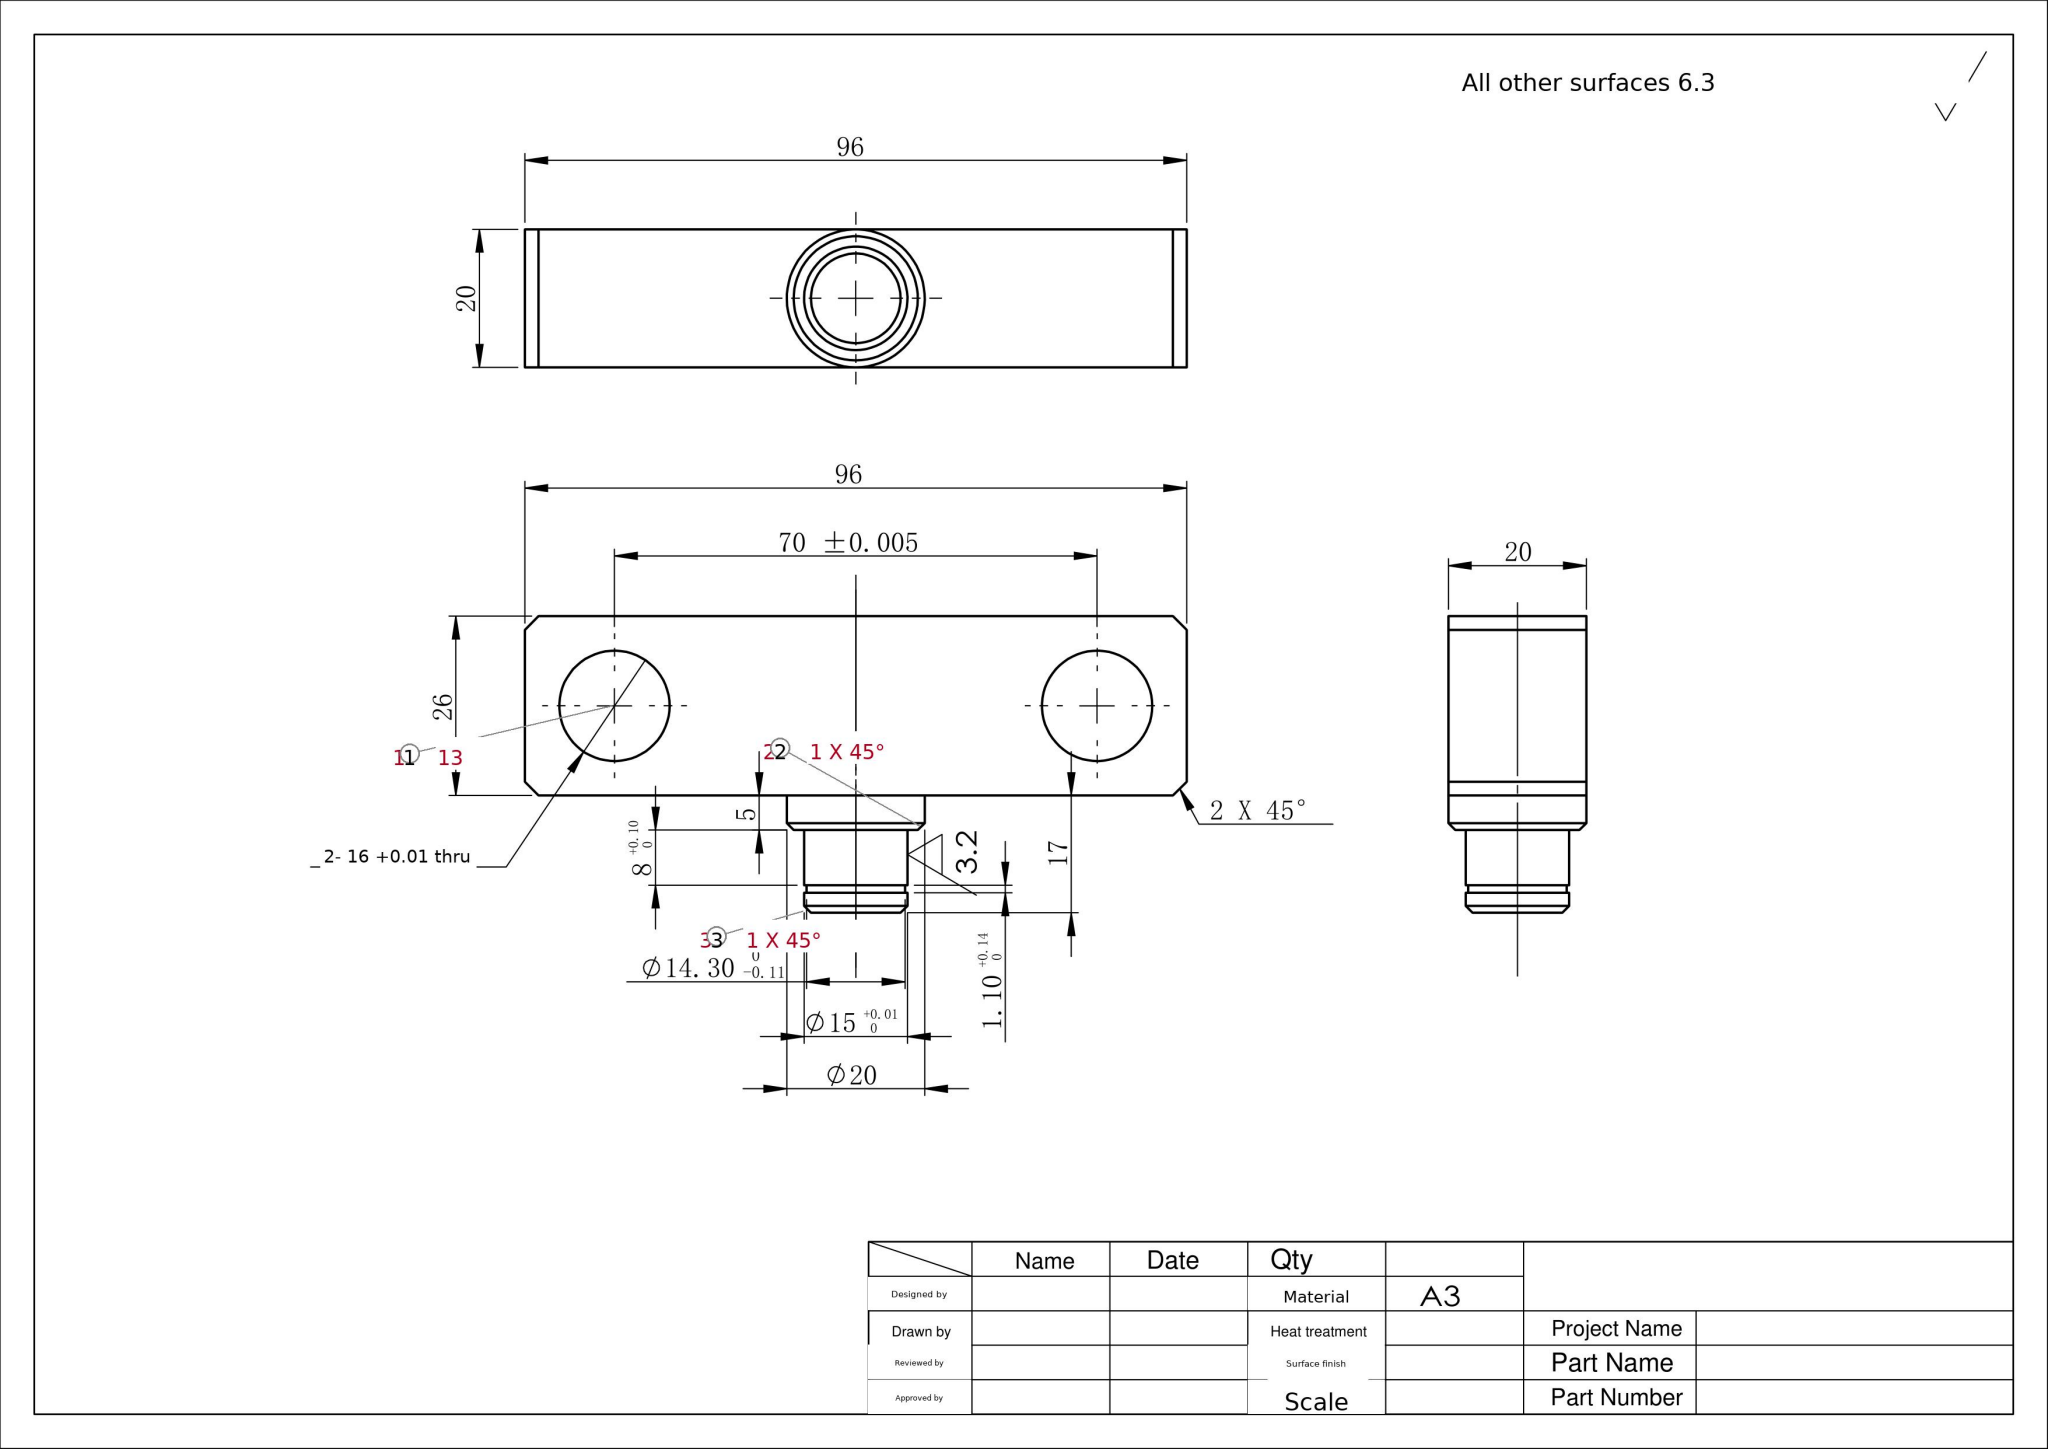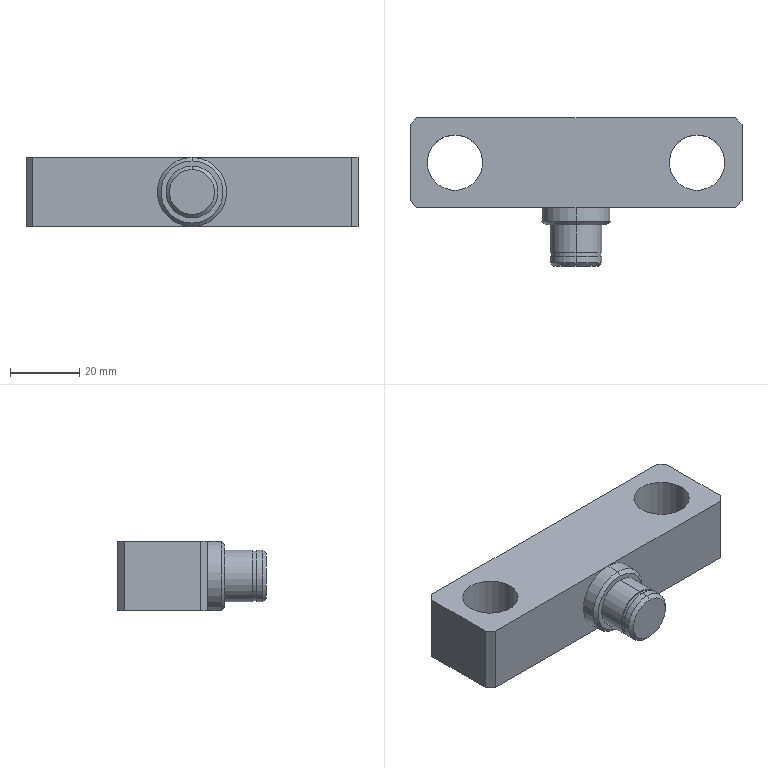Part | SolidWorks | mm | 1 solid | 31 faces | box 96 x 43 x 20 mm | volume 45338 mm3 | plane 15 | cylinder 12 | cone 4 | commonest cylinder face diameters 15 x4 16 x4 14.3 x2 20 x2
build123d program:
from build123d import *

# Parameters (mm, degrees)
SKETCH1_W      = 96
SKETCH1_H      = 26
SKETCH1_R      = 8
EXTRUDE1_DEPTH = 20
SKETCH2_R      = 10
EXTRUDE5_DEPTH = 5
SKETCH5_R      = 7.5
EXTRUDE6_DEPTH = 12
CHAMFER2_SIZE  = 1
SKETCH6_W      = 2.17
SKETCH6_H      = 1.1
CHAMFER3_SIZE  = 2


with BuildPart() as part:
    # Sketch1 → Extrude1 (new body)
    with BuildSketch(Plane.XY):
        with Locations((48, 13)):
            Rectangle(SKETCH1_W, SKETCH1_H)
        with Locations((13, 13)):
            Circle(SKETCH1_R, mode=Mode.SUBTRACT)
        with Locations((83, 13)):
            Circle(SKETCH1_R, mode=Mode.SUBTRACT)
    extrude(amount=EXTRUDE1_DEPTH)

    # Sketch2 → Extrude5 (add)
    with BuildSketch(Plane.XZ):
        with Locations(Location((48, 10, 0), (0, 0, 270))):
            Circle(SKETCH2_R)
    extrude(amount=EXTRUDE5_DEPTH)

    # Sketch5 → Extrude6 (add)
    with BuildSketch(Plane.XZ.offset(5)):
        with Locations(Location((48, 10, 0), (0, 0, 270))):
            Circle(SKETCH5_R)
    extrude(amount=EXTRUDE6_DEPTH)

    # Chamfer2
    chamfer2_edges = [part.edges().sort_by_distance(p)[0] for p in [
        (48, -5, 20),
        (48, -17, 17.5),
    ]]
    chamfer(chamfer2_edges, length=CHAMFER2_SIZE)

    # Sketch6 → Cut-Revolve1 (revolve, cut)
    with BuildSketch(Plane.XY.offset(10), mode=Mode.PRIVATE) as cut_revolve1_sk:
        with Locations((39.765, -13.55)):
            Rectangle(SKETCH6_W, SKETCH6_H)
    revolve(cut_revolve1_sk.sketch.rotate(Axis((48, -16, 10), (0, -1, 0)), 270), axis=Axis((48, -16, 10), (0, -1, 0)), mode=Mode.SUBTRACT)

    # Chamfer3
    chamfer3_edges = [part.edges().sort_by_distance(p)[0] for p in [
        (0, 26, 10),
        (96, 26, 10),
        (96, 0, 10),
        (0, 0, 10),
    ]]
    chamfer(chamfer3_edges, length=CHAMFER3_SIZE)


solid = part.part
STEP:
#1=CARTESIAN_POINT('',(48.,-16.,17.5));
#2=VERTEX_POINT('',#1);
#3=CARTESIAN_POINT('',(48.,-16.,2.5));
#4=VERTEX_POINT('',#3);
#5=CARTESIAN_POINT('',(48.,-16.,10.));
#6=DIRECTION('',(0.,1.,0.));
#7=DIRECTION('',(0.,0.,-1.));
#8=AXIS2_PLACEMENT_3D('',#5,#6,#7);
#9=CIRCLE('',#8,7.5);
#10=EDGE_CURVE('',#2,#4,#9,.T.);
#11=ORIENTED_EDGE('',*,*,#10,.T.);
#12=CARTESIAN_POINT('',(48.,-14.1,2.5));
#13=VERTEX_POINT('',#12);
#14=CARTESIAN_POINT('',(48.,-17.,2.5));
#15=DIRECTION('',(0.,1.,0.));
#16=VECTOR('',#15,1000.);
#17=LINE('',#14,#16);
#18=EDGE_CURVE('',#4,#13,#17,.T.);
#19=ORIENTED_EDGE('',*,*,#18,.T.);
#20=CARTESIAN_POINT('',(48.,-14.1,17.5));
#21=VERTEX_POINT('',#20);
#22=CARTESIAN_POINT('',(48.,-14.1,10.));
#23=DIRECTION('',(0.,-1.,0.));
#24=DIRECTION('',(0.,0.,-1.));
#25=AXIS2_PLACEMENT_3D('',#22,#23,#24);
#26=CIRCLE('',#25,7.5);
#27=EDGE_CURVE('',#13,#21,#26,.T.);
#28=ORIENTED_EDGE('',*,*,#27,.T.);
#29=CARTESIAN_POINT('',(48.,-17.,17.5));
#30=DIRECTION('',(0.,1.,0.));
#31=VECTOR('',#30,1000.);
#32=LINE('',#29,#31);
#33=EDGE_CURVE('',#2,#21,#32,.T.);
#34=ORIENTED_EDGE('',*,*,#33,.F.);
#35=EDGE_LOOP('',(#11,#19,#28,#34));
#36=FACE_OUTER_BOUND('',#35,.T.);
#37=CARTESIAN_POINT('',(48.,-17.,10.));
#38=DIRECTION('',(0.,1.,0.));
#39=DIRECTION('',(0.,0.,1.));
#40=AXIS2_PLACEMENT_3D('',#37,#38,#39);
#41=CYLINDRICAL_SURFACE('',#40,7.5);
#42=ADVANCED_FACE('',(#36),#41,.T.);
#43=CARTESIAN_POINT('',(48.,-17.,3.5));
#44=VERTEX_POINT('',#43);
#45=CARTESIAN_POINT('',(48.,-17.,16.5));
#46=VERTEX_POINT('',#45);
#47=CARTESIAN_POINT('',(48.,-17.,10.));
#48=DIRECTION('',(0.,-1.,0.));
#49=DIRECTION('',(0.,0.,-1.));
#50=AXIS2_PLACEMENT_3D('',#47,#48,#49);
#51=CIRCLE('',#50,6.5);
#52=EDGE_CURVE('',#44,#46,#51,.T.);
#53=ORIENTED_EDGE('',*,*,#52,.F.);
#54=CARTESIAN_POINT('',(48.,-17.,3.5));
#55=DIRECTION('',(0.,0.7071,-0.7071));
#56=VECTOR('',#55,1000.);
#57=LINE('',#54,#56);
#58=EDGE_CURVE('',#44,#4,#57,.T.);
#59=ORIENTED_EDGE('',*,*,#58,.T.);
#60=ORIENTED_EDGE('',*,*,#10,.F.);
#61=CARTESIAN_POINT('',(48.,-17.,16.5));
#62=DIRECTION('',(0.,0.7071,0.7071));
#63=VECTOR('',#62,1000.);
#64=LINE('',#61,#63);
#65=EDGE_CURVE('',#46,#2,#64,.T.);
#66=ORIENTED_EDGE('',*,*,#65,.F.);
#67=EDGE_LOOP('',(#53,#59,#60,#66));
#68=FACE_OUTER_BOUND('',#67,.T.);
#69=CARTESIAN_POINT('',(48.,-17.,10.));
#70=DIRECTION('',(0.,1.,0.));
#71=DIRECTION('',(0.,0.,1.));
#72=AXIS2_PLACEMENT_3D('',#69,#70,#71);
#73=CONICAL_SURFACE('',#72,6.5,0.7854);
#74=ADVANCED_FACE('',(#68),#73,.T.);
#75=CARTESIAN_POINT('',(48.,-14.1,17.15));
#76=VERTEX_POINT('',#75);
#77=CARTESIAN_POINT('',(48.,-14.1,2.85));
#78=VERTEX_POINT('',#77);
#79=CARTESIAN_POINT('',(48.,-14.1,10.));
#80=DIRECTION('',(0.,1.,0.));
#81=DIRECTION('',(0.,0.,1.));
#82=AXIS2_PLACEMENT_3D('',#79,#80,#81);
#83=CIRCLE('',#82,7.15);
#84=EDGE_CURVE('',#76,#78,#83,.T.);
#85=ORIENTED_EDGE('',*,*,#84,.T.);
#86=CARTESIAN_POINT('',(48.,-13.,2.85));
#87=VERTEX_POINT('',#86);
#88=CARTESIAN_POINT('',(48.,-16.,2.85));
#89=DIRECTION('',(0.,1.,0.));
#90=VECTOR('',#89,1000.);
#91=LINE('',#88,#90);
#92=EDGE_CURVE('',#78,#87,#91,.T.);
#93=ORIENTED_EDGE('',*,*,#92,.T.);
#94=CARTESIAN_POINT('',(48.,-13.,17.15));
#95=VERTEX_POINT('',#94);
#96=CARTESIAN_POINT('',(48.,-13.,10.));
#97=DIRECTION('',(0.,1.,0.));
#98=DIRECTION('',(0.,0.,1.));
#99=AXIS2_PLACEMENT_3D('',#96,#97,#98);
#100=CIRCLE('',#99,7.15);
#101=EDGE_CURVE('',#95,#87,#100,.T.);
#102=ORIENTED_EDGE('',*,*,#101,.F.);
#103=CARTESIAN_POINT('',(48.,-16.,17.15));
#104=DIRECTION('',(0.,1.,0.));
#105=VECTOR('',#104,1000.);
#106=LINE('',#103,#105);
#107=EDGE_CURVE('',#76,#95,#106,.T.);
#108=ORIENTED_EDGE('',*,*,#107,.F.);
#109=EDGE_LOOP('',(#85,#93,#102,#108));
#110=FACE_OUTER_BOUND('',#109,.T.);
#111=CARTESIAN_POINT('',(48.,-16.,10.));
#112=DIRECTION('',(0.,1.,0.));
#113=DIRECTION('',(0.,0.,1.));
#114=AXIS2_PLACEMENT_3D('',#111,#112,#113);
#115=CYLINDRICAL_SURFACE('',#114,7.15);
#116=ADVANCED_FACE('',(#110),#115,.T.);
#117=CARTESIAN_POINT('',(48.,-5.,1.));
#118=VERTEX_POINT('',#117);
#119=CARTESIAN_POINT('',(48.,-5.,19.));
#120=VERTEX_POINT('',#119);
#121=CARTESIAN_POINT('',(48.,-5.,10.));
#122=DIRECTION('',(0.,-1.,0.));
#123=DIRECTION('',(0.,0.,-1.));
#124=AXIS2_PLACEMENT_3D('',#121,#122,#123);
#125=CIRCLE('',#124,9.);
#126=EDGE_CURVE('',#118,#120,#125,.T.);
#127=ORIENTED_EDGE('',*,*,#126,.F.);
#128=CARTESIAN_POINT('',(48.,-4.,-0.));
#129=VERTEX_POINT('',#128);
#130=CARTESIAN_POINT('',(48.,-5.,1.));
#131=DIRECTION('',(0.,0.7071,-0.7071));
#132=VECTOR('',#131,1000.);
#133=LINE('',#130,#132);
#134=EDGE_CURVE('',#118,#129,#133,.T.);
#135=ORIENTED_EDGE('',*,*,#134,.T.);
#136=CARTESIAN_POINT('',(48.,-4.,20.));
#137=VERTEX_POINT('',#136);
#138=CARTESIAN_POINT('',(48.,-4.,10.));
#139=DIRECTION('',(0.,1.,0.));
#140=DIRECTION('',(0.,0.,-1.));
#141=AXIS2_PLACEMENT_3D('',#138,#139,#140);
#142=CIRCLE('',#141,10.);
#143=EDGE_CURVE('',#137,#129,#142,.T.);
#144=ORIENTED_EDGE('',*,*,#143,.F.);
#145=CARTESIAN_POINT('',(48.,-5.,19.));
#146=DIRECTION('',(0.,0.7071,0.7071));
#147=VECTOR('',#146,1000.);
#148=LINE('',#145,#147);
#149=EDGE_CURVE('',#120,#137,#148,.T.);
#150=ORIENTED_EDGE('',*,*,#149,.F.);
#151=EDGE_LOOP('',(#127,#135,#144,#150));
#152=FACE_OUTER_BOUND('',#151,.T.);
#153=CARTESIAN_POINT('',(48.,-5.,10.));
#154=DIRECTION('',(0.,1.,0.));
#155=DIRECTION('',(0.,0.,1.));
#156=AXIS2_PLACEMENT_3D('',#153,#154,#155);
#157=CONICAL_SURFACE('',#156,9.,0.7854);
#158=ADVANCED_FACE('',(#152),#157,.T.);
#159=ORIENTED_EDGE('',*,*,#143,.T.);
#160=CARTESIAN_POINT('',(48.,0.,-0.));
#161=VERTEX_POINT('',#160);
#162=CARTESIAN_POINT('',(48.,-5.,-0.));
#163=DIRECTION('',(0.,1.,0.));
#164=VECTOR('',#163,1000.);
#165=LINE('',#162,#164);
#166=EDGE_CURVE('',#129,#161,#165,.T.);
#167=ORIENTED_EDGE('',*,*,#166,.T.);
#168=CARTESIAN_POINT('',(48.,0.,20.));
#169=VERTEX_POINT('',#168);
#170=CARTESIAN_POINT('',(48.,0.,10.));
#171=DIRECTION('',(0.,-1.,0.));
#172=DIRECTION('',(0.,0.,-1.));
#173=AXIS2_PLACEMENT_3D('',#170,#171,#172);
#174=CIRCLE('',#173,10.);
#175=EDGE_CURVE('',#161,#169,#174,.T.);
#176=ORIENTED_EDGE('',*,*,#175,.T.);
#177=CARTESIAN_POINT('',(48.,-5.,20.));
#178=DIRECTION('',(0.,1.,0.));
#179=VECTOR('',#178,1000.);
#180=LINE('',#177,#179);
#181=EDGE_CURVE('',#137,#169,#180,.T.);
#182=ORIENTED_EDGE('',*,*,#181,.F.);
#183=EDGE_LOOP('',(#159,#167,#176,#182));
#184=FACE_OUTER_BOUND('',#183,.T.);
#185=CARTESIAN_POINT('',(48.,-5.,10.));
#186=DIRECTION('',(0.,1.,0.));
#187=DIRECTION('',(0.,0.,1.));
#188=AXIS2_PLACEMENT_3D('',#185,#186,#187);
#189=CYLINDRICAL_SURFACE('',#188,10.);
#190=ADVANCED_FACE('',(#184),#189,.T.);
#191=CARTESIAN_POINT('',(75.,13.,20.));
#192=VERTEX_POINT('',#191);
#193=CARTESIAN_POINT('',(91.,13.,20.));
#194=VERTEX_POINT('',#193);
#195=CARTESIAN_POINT('',(83.,13.,20.));
#196=DIRECTION('',(0.,0.,1.));
#197=DIRECTION('',(1.,0.,0.));
#198=AXIS2_PLACEMENT_3D('',#195,#196,#197);
#199=CIRCLE('',#198,8.);
#200=EDGE_CURVE('',#192,#194,#199,.T.);
#201=ORIENTED_EDGE('',*,*,#200,.T.);
#202=CARTESIAN_POINT('',(91.,13.,0.));
#203=VERTEX_POINT('',#202);
#204=CARTESIAN_POINT('',(91.,13.,20.));
#205=DIRECTION('',(0.,0.,-1.));
#206=VECTOR('',#205,1000.);
#207=LINE('',#204,#206);
#208=EDGE_CURVE('',#194,#203,#207,.T.);
#209=ORIENTED_EDGE('',*,*,#208,.T.);
#210=CARTESIAN_POINT('',(75.,13.,0.));
#211=VERTEX_POINT('',#210);
#212=CARTESIAN_POINT('',(83.,13.,0.));
#213=DIRECTION('',(0.,0.,1.));
#214=DIRECTION('',(1.,0.,0.));
#215=AXIS2_PLACEMENT_3D('',#212,#213,#214);
#216=CIRCLE('',#215,8.);
#217=EDGE_CURVE('',#211,#203,#216,.T.);
#218=ORIENTED_EDGE('',*,*,#217,.F.);
#219=CARTESIAN_POINT('',(75.,13.,20.));
#220=DIRECTION('',(0.,0.,-1.));
#221=VECTOR('',#220,1000.);
#222=LINE('',#219,#221);
#223=EDGE_CURVE('',#192,#211,#222,.T.);
#224=ORIENTED_EDGE('',*,*,#223,.F.);
#225=EDGE_LOOP('',(#201,#209,#218,#224));
#226=FACE_OUTER_BOUND('',#225,.T.);
#227=CARTESIAN_POINT('',(83.,13.,20.));
#228=DIRECTION('',(0.,0.,-1.));
#229=DIRECTION('',(-1.,0.,0.));
#230=AXIS2_PLACEMENT_3D('',#227,#228,#229);
#231=CYLINDRICAL_SURFACE('',#230,8.);
#232=ADVANCED_FACE('',(#226),#231,.F.);
#233=CARTESIAN_POINT('',(5.,13.,20.));
#234=VERTEX_POINT('',#233);
#235=CARTESIAN_POINT('',(21.,13.,20.));
#236=VERTEX_POINT('',#235);
#237=CARTESIAN_POINT('',(13.,13.,20.));
#238=DIRECTION('',(0.,0.,1.));
#239=DIRECTION('',(1.,0.,0.));
#240=AXIS2_PLACEMENT_3D('',#237,#238,#239);
#241=CIRCLE('',#240,8.);
#242=EDGE_CURVE('',#234,#236,#241,.T.);
#243=ORIENTED_EDGE('',*,*,#242,.T.);
#244=CARTESIAN_POINT('',(21.,13.,0.));
#245=VERTEX_POINT('',#244);
#246=CARTESIAN_POINT('',(21.,13.,20.));
#247=DIRECTION('',(0.,0.,-1.));
#248=VECTOR('',#247,1000.);
#249=LINE('',#246,#248);
#250=EDGE_CURVE('',#236,#245,#249,.T.);
#251=ORIENTED_EDGE('',*,*,#250,.T.);
#252=CARTESIAN_POINT('',(5.,13.,0.));
#253=VERTEX_POINT('',#252);
#254=CARTESIAN_POINT('',(13.,13.,0.));
#255=DIRECTION('',(0.,0.,1.));
#256=DIRECTION('',(1.,0.,0.));
#257=AXIS2_PLACEMENT_3D('',#254,#255,#256);
#258=CIRCLE('',#257,8.);
#259=EDGE_CURVE('',#253,#245,#258,.T.);
#260=ORIENTED_EDGE('',*,*,#259,.F.);
#261=CARTESIAN_POINT('',(5.,13.,20.));
#262=DIRECTION('',(0.,0.,-1.));
#263=VECTOR('',#262,1000.);
#264=LINE('',#261,#263);
#265=EDGE_CURVE('',#234,#253,#264,.T.);
#266=ORIENTED_EDGE('',*,*,#265,.F.);
#267=EDGE_LOOP('',(#243,#251,#260,#266));
#268=FACE_OUTER_BOUND('',#267,.T.);
#269=CARTESIAN_POINT('',(13.,13.,20.));
#270=DIRECTION('',(0.,0.,-1.));
#271=DIRECTION('',(-1.,0.,0.));
#272=AXIS2_PLACEMENT_3D('',#269,#270,#271);
#273=CYLINDRICAL_SURFACE('',#272,8.);
#274=ADVANCED_FACE('',(#268),#273,.F.);
#275=CARTESIAN_POINT('',(48.,-13.,17.5));
#276=VERTEX_POINT('',#275);
#277=CARTESIAN_POINT('',(48.,-13.,2.5));
#278=VERTEX_POINT('',#277);
#279=CARTESIAN_POINT('',(48.,-13.,10.));
#280=DIRECTION('',(0.,1.,0.));
#281=DIRECTION('',(0.,0.,1.));
#282=AXIS2_PLACEMENT_3D('',#279,#280,#281);
#283=CIRCLE('',#282,7.5);
#284=EDGE_CURVE('',#276,#278,#283,.T.);
#285=ORIENTED_EDGE('',*,*,#284,.T.);
#286=CARTESIAN_POINT('',(48.,-5.,2.5));
#287=VERTEX_POINT('',#286);
#288=CARTESIAN_POINT('',(48.,-17.,2.5));
#289=DIRECTION('',(0.,1.,0.));
#290=VECTOR('',#289,1000.);
#291=LINE('',#288,#290);
#292=EDGE_CURVE('',#278,#287,#291,.T.);
#293=ORIENTED_EDGE('',*,*,#292,.T.);
#294=CARTESIAN_POINT('',(48.,-5.,17.5));
#295=VERTEX_POINT('',#294);
#296=CARTESIAN_POINT('',(48.,-5.,10.));
#297=DIRECTION('',(0.,-1.,0.));
#298=DIRECTION('',(0.,0.,-1.));
#299=AXIS2_PLACEMENT_3D('',#296,#297,#298);
#300=CIRCLE('',#299,7.5);
#301=EDGE_CURVE('',#287,#295,#300,.T.);
#302=ORIENTED_EDGE('',*,*,#301,.T.);
#303=CARTESIAN_POINT('',(48.,-17.,17.5));
#304=DIRECTION('',(0.,1.,0.));
#305=VECTOR('',#304,1000.);
#306=LINE('',#303,#305);
#307=EDGE_CURVE('',#276,#295,#306,.T.);
#308=ORIENTED_EDGE('',*,*,#307,.F.);
#309=EDGE_LOOP('',(#285,#293,#302,#308));
#310=FACE_OUTER_BOUND('',#309,.T.);
#311=CARTESIAN_POINT('',(48.,-17.,10.));
#312=DIRECTION('',(0.,1.,0.));
#313=DIRECTION('',(0.,0.,1.));
#314=AXIS2_PLACEMENT_3D('',#311,#312,#313);
#315=CYLINDRICAL_SURFACE('',#314,7.5);
#316=ADVANCED_FACE('',(#310),#315,.T.);
#317=ORIENTED_EDGE('',*,*,#292,.F.);
#318=CARTESIAN_POINT('',(48.,-13.,10.));
#319=DIRECTION('',(0.,1.,0.));
#320=DIRECTION('',(0.,0.,1.));
#321=AXIS2_PLACEMENT_3D('',#318,#319,#320);
#322=CIRCLE('',#321,7.5);
#323=EDGE_CURVE('',#278,#276,#322,.T.);
#324=ORIENTED_EDGE('',*,*,#323,.T.);
#325=ORIENTED_EDGE('',*,*,#307,.T.);
#326=CARTESIAN_POINT('',(48.,-5.,10.));
#327=DIRECTION('',(0.,-1.,0.));
#328=DIRECTION('',(0.,0.,-1.));
#329=AXIS2_PLACEMENT_3D('',#326,#327,#328);
#330=CIRCLE('',#329,7.5);
#331=EDGE_CURVE('',#295,#287,#330,.T.);
#332=ORIENTED_EDGE('',*,*,#331,.T.);
#333=EDGE_LOOP('',(#317,#324,#325,#332));
#334=FACE_OUTER_BOUND('',#333,.T.);
#335=CARTESIAN_POINT('',(48.,-17.,10.));
#336=DIRECTION('',(0.,1.,0.));
#337=DIRECTION('',(0.,0.,1.));
#338=AXIS2_PLACEMENT_3D('',#335,#336,#337);
#339=CYLINDRICAL_SURFACE('',#338,7.5);
#340=ADVANCED_FACE('',(#334),#339,.T.);
#341=CARTESIAN_POINT('',(48.,-5.,10.));
#342=DIRECTION('',(0.,-1.,0.));
#343=DIRECTION('',(0.,0.,-1.));
#344=AXIS2_PLACEMENT_3D('',#341,#342,#343);
#345=CIRCLE('',#344,9.);
#346=EDGE_CURVE('',#120,#118,#345,.T.);
#347=ORIENTED_EDGE('',*,*,#346,.T.);
#348=ORIENTED_EDGE('',*,*,#126,.T.);
#349=EDGE_LOOP('',(#347,#348));
#350=FACE_OUTER_BOUND('',#349,.T.);
#351=ORIENTED_EDGE('',*,*,#331,.F.);
#352=ORIENTED_EDGE('',*,*,#301,.F.);
#353=EDGE_LOOP('',(#351,#352));
#354=FACE_BOUND('',#353,.T.);
#355=CARTESIAN_POINT('',(48.,-5.,10.));
#356=DIRECTION('',(0.,-1.,0.));
#357=DIRECTION('',(0.,0.,-1.));
#358=AXIS2_PLACEMENT_3D('',#355,#356,#357);
#359=PLANE('',#358);
#360=ADVANCED_FACE('',(#350,#354),#359,.T.);
#361=CARTESIAN_POINT('',(94.,0.,0.));
#362=VERTEX_POINT('',#361);
#363=CARTESIAN_POINT('',(0.,0.,0.));
#364=DIRECTION('',(1.,0.,0.));
#365=VECTOR('',#364,1000.);
#366=LINE('',#363,#365);
#367=EDGE_CURVE('',#161,#362,#366,.T.);
#368=ORIENTED_EDGE('',*,*,#367,.T.);
#369=CARTESIAN_POINT('',(94.,-0.,20.));
#370=VERTEX_POINT('',#369);
#371=CARTESIAN_POINT('',(94.,0.,20.));
#372=DIRECTION('',(0.,0.,1.));
#373=VECTOR('',#372,1000.);
#374=LINE('',#371,#373);
#375=EDGE_CURVE('',#362,#370,#374,.T.);
#376=ORIENTED_EDGE('',*,*,#375,.T.);
#377=CARTESIAN_POINT('',(0.,0.,20.));
#378=DIRECTION('',(1.,0.,0.));
#379=VECTOR('',#378,1000.);
#380=LINE('',#377,#379);
#381=EDGE_CURVE('',#169,#370,#380,.T.);
#382=ORIENTED_EDGE('',*,*,#381,.F.);
#383=ORIENTED_EDGE('',*,*,#175,.F.);
#384=EDGE_LOOP('',(#368,#376,#382,#383));
#385=FACE_OUTER_BOUND('',#384,.T.);
#386=CARTESIAN_POINT('',(0.,0.,20.));
#387=DIRECTION('',(0.,1.,0.));
#388=DIRECTION('',(0.,0.,1.));
#389=AXIS2_PLACEMENT_3D('',#386,#387,#388);
#390=PLANE('',#389);
#391=ADVANCED_FACE('',(#385),#390,.F.);
#392=CARTESIAN_POINT('',(2.,0.,20.));
#393=VERTEX_POINT('',#392);
#394=CARTESIAN_POINT('',(0.,0.,20.));
#395=DIRECTION('',(1.,0.,0.));
#396=VECTOR('',#395,1000.);
#397=LINE('',#394,#396);
#398=EDGE_CURVE('',#393,#169,#397,.T.);
#399=ORIENTED_EDGE('',*,*,#398,.F.);
#400=CARTESIAN_POINT('',(2.,0.,0.));
#401=VERTEX_POINT('',#400);
#402=CARTESIAN_POINT('',(2.,0.,20.));
#403=DIRECTION('',(0.,0.,-1.));
#404=VECTOR('',#403,1000.);
#405=LINE('',#402,#404);
#406=EDGE_CURVE('',#393,#401,#405,.T.);
#407=ORIENTED_EDGE('',*,*,#406,.T.);
#408=CARTESIAN_POINT('',(0.,0.,0.));
#409=DIRECTION('',(1.,0.,0.));
#410=VECTOR('',#409,1000.);
#411=LINE('',#408,#410);
#412=EDGE_CURVE('',#401,#161,#411,.T.);
#413=ORIENTED_EDGE('',*,*,#412,.T.);
#414=CARTESIAN_POINT('',(48.,0.,10.));
#415=DIRECTION('',(0.,-1.,0.));
#416=DIRECTION('',(0.,0.,-1.));
#417=AXIS2_PLACEMENT_3D('',#414,#415,#416);
#418=CIRCLE('',#417,10.);
#419=EDGE_CURVE('',#169,#161,#418,.T.);
#420=ORIENTED_EDGE('',*,*,#419,.F.);
#421=EDGE_LOOP('',(#399,#407,#413,#420));
#422=FACE_OUTER_BOUND('',#421,.T.);
#423=CARTESIAN_POINT('',(0.,0.,20.));
#424=DIRECTION('',(0.,1.,0.));
#425=DIRECTION('',(0.,0.,1.));
#426=AXIS2_PLACEMENT_3D('',#423,#424,#425);
#427=PLANE('',#426);
#428=ADVANCED_FACE('',(#422),#427,.F.);
#429=ORIENTED_EDGE('',*,*,#242,.F.);
#430=CARTESIAN_POINT('',(13.,13.,20.));
#431=DIRECTION('',(0.,0.,1.));
#432=DIRECTION('',(1.,0.,0.));
#433=AXIS2_PLACEMENT_3D('',#430,#431,#432);
#434=CIRCLE('',#433,8.);
#435=EDGE_CURVE('',#236,#234,#434,.T.);
#436=ORIENTED_EDGE('',*,*,#435,.F.);
#437=EDGE_LOOP('',(#429,#436));
#438=FACE_BOUND('',#437,.T.);
#439=CARTESIAN_POINT('',(96.,2.,20.));
#440=VERTEX_POINT('',#439);
#441=CARTESIAN_POINT('',(96.,24.,20.));
#442=VERTEX_POINT('',#441);
#443=CARTESIAN_POINT('',(96.,0.,20.));
#444=DIRECTION('',(0.,1.,0.));
#445=VECTOR('',#444,1000.);
#446=LINE('',#443,#445);
#447=EDGE_CURVE('',#440,#442,#446,.T.);
#448=ORIENTED_EDGE('',*,*,#447,.T.);
#449=CARTESIAN_POINT('',(94.,26.,20.));
#450=VERTEX_POINT('',#449);
#451=CARTESIAN_POINT('',(94.,26.,20.));
#452=DIRECTION('',(-0.7071,0.7071,0.));
#453=VECTOR('',#452,1000.);
#454=LINE('',#451,#453);
#455=EDGE_CURVE('',#442,#450,#454,.T.);
#456=ORIENTED_EDGE('',*,*,#455,.T.);
#457=CARTESIAN_POINT('',(2.,26.,20.));
#458=VERTEX_POINT('',#457);
#459=CARTESIAN_POINT('',(0.,26.,20.));
#460=DIRECTION('',(-1.,0.,0.));
#461=VECTOR('',#460,1000.);
#462=LINE('',#459,#461);
#463=EDGE_CURVE('',#450,#458,#462,.T.);
#464=ORIENTED_EDGE('',*,*,#463,.T.);
#465=CARTESIAN_POINT('',(-0.,24.,20.));
#466=VERTEX_POINT('',#465);
#467=CARTESIAN_POINT('',(0.,24.,20.));
#468=DIRECTION('',(-0.7071,-0.7071,0.));
#469=VECTOR('',#468,1000.);
#470=LINE('',#467,#469);
#471=EDGE_CURVE('',#458,#466,#470,.T.);
#472=ORIENTED_EDGE('',*,*,#471,.T.);
#473=CARTESIAN_POINT('',(-0.,2.,20.));
#474=VERTEX_POINT('',#473);
#475=CARTESIAN_POINT('',(0.,0.,20.));
#476=DIRECTION('',(0.,-1.,0.));
#477=VECTOR('',#476,1000.);
#478=LINE('',#475,#477);
#479=EDGE_CURVE('',#466,#474,#478,.T.);
#480=ORIENTED_EDGE('',*,*,#479,.T.);
#481=CARTESIAN_POINT('',(2.,0.,20.));
#482=DIRECTION('',(0.7071,-0.7071,0.));
#483=VECTOR('',#482,1000.);
#484=LINE('',#481,#483);
#485=EDGE_CURVE('',#474,#393,#484,.T.);
#486=ORIENTED_EDGE('',*,*,#485,.T.);
#487=ORIENTED_EDGE('',*,*,#398,.T.);
#488=ORIENTED_EDGE('',*,*,#381,.T.);
#489=CARTESIAN_POINT('',(96.,2.,20.));
#490=DIRECTION('',(0.7071,0.7071,0.));
#491=VECTOR('',#490,1000.);
#492=LINE('',#489,#491);
#493=EDGE_CURVE('',#370,#440,#492,.T.);
#494=ORIENTED_EDGE('',*,*,#493,.T.);
#495=EDGE_LOOP('',(#448,#456,#464,#472,#480,#486,#487,#488,#494));
#496=FACE_OUTER_BOUND('',#495,.T.);
#497=ORIENTED_EDGE('',*,*,#200,.F.);
#498=CARTESIAN_POINT('',(83.,13.,20.));
#499=DIRECTION('',(0.,0.,1.));
#500=DIRECTION('',(1.,0.,0.));
#501=AXIS2_PLACEMENT_3D('',#498,#499,#500);
#502=CIRCLE('',#501,8.);
#503=EDGE_CURVE('',#194,#192,#502,.T.);
#504=ORIENTED_EDGE('',*,*,#503,.F.);
#505=EDGE_LOOP('',(#497,#504));
#506=FACE_BOUND('',#505,.T.);
#507=CARTESIAN_POINT('',(0.,0.,20.));
#508=DIRECTION('',(0.,0.,-1.));
#509=DIRECTION('',(-1.,0.,0.));
#510=AXIS2_PLACEMENT_3D('',#507,#508,#509);
#511=PLANE('',#510);
#512=ADVANCED_FACE('',(#438,#496,#506),#511,.F.);
#513=ORIENTED_EDGE('',*,*,#259,.T.);
#514=CARTESIAN_POINT('',(13.,13.,0.));
#515=DIRECTION('',(0.,0.,1.));
#516=DIRECTION('',(1.,0.,0.));
#517=AXIS2_PLACEMENT_3D('',#514,#515,#516);
#518=CIRCLE('',#517,8.);
#519=EDGE_CURVE('',#245,#253,#518,.T.);
#520=ORIENTED_EDGE('',*,*,#519,.T.);
#521=EDGE_LOOP('',(#513,#520));
#522=FACE_BOUND('',#521,.T.);
#523=CARTESIAN_POINT('',(94.,26.,0.));
#524=VERTEX_POINT('',#523);
#525=CARTESIAN_POINT('',(2.,26.,0.));
#526=VERTEX_POINT('',#525);
#527=CARTESIAN_POINT('',(0.,26.,0.));
#528=DIRECTION('',(-1.,0.,0.));
#529=VECTOR('',#528,1000.);
#530=LINE('',#527,#529);
#531=EDGE_CURVE('',#524,#526,#530,.T.);
#532=ORIENTED_EDGE('',*,*,#531,.F.);
#533=CARTESIAN_POINT('',(96.,24.,0.));
#534=VERTEX_POINT('',#533);
#535=CARTESIAN_POINT('',(60.,60.,0.));
#536=DIRECTION('',(0.7071,-0.7071,0.));
#537=VECTOR('',#536,1000.);
#538=LINE('',#535,#537);
#539=EDGE_CURVE('',#524,#534,#538,.T.);
#540=ORIENTED_EDGE('',*,*,#539,.T.);
#541=CARTESIAN_POINT('',(96.,2.,0.));
#542=VERTEX_POINT('',#541);
#543=CARTESIAN_POINT('',(96.,0.,0.));
#544=DIRECTION('',(0.,1.,0.));
#545=VECTOR('',#544,1000.);
#546=LINE('',#543,#545);
#547=EDGE_CURVE('',#542,#534,#546,.T.);
#548=ORIENTED_EDGE('',*,*,#547,.F.);
#549=CARTESIAN_POINT('',(47.,-47.,0.));
#550=DIRECTION('',(-0.7071,-0.7071,0.));
#551=VECTOR('',#550,1000.);
#552=LINE('',#549,#551);
#553=EDGE_CURVE('',#542,#362,#552,.T.);
#554=ORIENTED_EDGE('',*,*,#553,.T.);
#555=ORIENTED_EDGE('',*,*,#367,.F.);
#556=ORIENTED_EDGE('',*,*,#412,.F.);
#557=CARTESIAN_POINT('',(0.,2.,0.));
#558=VERTEX_POINT('',#557);
#559=CARTESIAN_POINT('',(1.,1.,0.));
#560=DIRECTION('',(-0.7071,0.7071,0.));
#561=VECTOR('',#560,1000.);
#562=LINE('',#559,#561);
#563=EDGE_CURVE('',#401,#558,#562,.T.);
#564=ORIENTED_EDGE('',*,*,#563,.T.);
#565=CARTESIAN_POINT('',(0.,24.,0.));
#566=VERTEX_POINT('',#565);
#567=CARTESIAN_POINT('',(0.,0.,0.));
#568=DIRECTION('',(0.,-1.,0.));
#569=VECTOR('',#568,1000.);
#570=LINE('',#567,#569);
#571=EDGE_CURVE('',#566,#558,#570,.T.);
#572=ORIENTED_EDGE('',*,*,#571,.F.);
#573=CARTESIAN_POINT('',(-12.,12.,0.));
#574=DIRECTION('',(0.7071,0.7071,0.));
#575=VECTOR('',#574,1000.);
#576=LINE('',#573,#575);
#577=EDGE_CURVE('',#566,#526,#576,.T.);
#578=ORIENTED_EDGE('',*,*,#577,.T.);
#579=EDGE_LOOP('',(#532,#540,#548,#554,#555,#556,#564,#572,#578));
#580=FACE_OUTER_BOUND('',#579,.T.);
#581=ORIENTED_EDGE('',*,*,#217,.T.);
#582=CARTESIAN_POINT('',(83.,13.,0.));
#583=DIRECTION('',(0.,0.,1.));
#584=DIRECTION('',(1.,0.,0.));
#585=AXIS2_PLACEMENT_3D('',#582,#583,#584);
#586=CIRCLE('',#585,8.);
#587=EDGE_CURVE('',#203,#211,#586,.T.);
#588=ORIENTED_EDGE('',*,*,#587,.T.);
#589=EDGE_LOOP('',(#581,#588));
#590=FACE_BOUND('',#589,.T.);
#591=CARTESIAN_POINT('',(0.,0.,0.));
#592=DIRECTION('',(0.,0.,-1.));
#593=DIRECTION('',(-1.,0.,0.));
#594=AXIS2_PLACEMENT_3D('',#591,#592,#593);
#595=PLANE('',#594);
#596=ADVANCED_FACE('',(#522,#580,#590),#595,.T.);
#597=ORIENTED_EDGE('',*,*,#479,.F.);
#598=CARTESIAN_POINT('',(0.,24.,20.));
#599=DIRECTION('',(0.,0.,-1.));
#600=VECTOR('',#599,1000.);
#601=LINE('',#598,#600);
#602=EDGE_CURVE('',#466,#566,#601,.T.);
#603=ORIENTED_EDGE('',*,*,#602,.T.);
#604=ORIENTED_EDGE('',*,*,#571,.T.);
#605=CARTESIAN_POINT('',(0.,2.,20.));
#606=DIRECTION('',(0.,0.,1.));
#607=VECTOR('',#606,1000.);
#608=LINE('',#605,#607);
#609=EDGE_CURVE('',#558,#474,#608,.T.);
#610=ORIENTED_EDGE('',*,*,#609,.T.);
#611=EDGE_LOOP('',(#597,#603,#604,#610));
#612=FACE_OUTER_BOUND('',#611,.T.);
#613=CARTESIAN_POINT('',(0.,0.,20.));
#614=DIRECTION('',(1.,0.,0.));
#615=DIRECTION('',(0.,0.,-1.));
#616=AXIS2_PLACEMENT_3D('',#613,#614,#615);
#617=PLANE('',#616);
#618=ADVANCED_FACE('',(#612),#617,.F.);
#619=ORIENTED_EDGE('',*,*,#547,.T.);
#620=CARTESIAN_POINT('',(96.,24.,20.));
#621=DIRECTION('',(0.,0.,1.));
#622=VECTOR('',#621,1000.);
#623=LINE('',#620,#622);
#624=EDGE_CURVE('',#534,#442,#623,.T.);
#625=ORIENTED_EDGE('',*,*,#624,.T.);
#626=ORIENTED_EDGE('',*,*,#447,.F.);
#627=CARTESIAN_POINT('',(96.,2.,20.));
#628=DIRECTION('',(0.,0.,-1.));
#629=VECTOR('',#628,1000.);
#630=LINE('',#627,#629);
#631=EDGE_CURVE('',#440,#542,#630,.T.);
#632=ORIENTED_EDGE('',*,*,#631,.T.);
#633=EDGE_LOOP('',(#619,#625,#626,#632));
#634=FACE_OUTER_BOUND('',#633,.T.);
#635=CARTESIAN_POINT('',(96.,0.,20.));
#636=DIRECTION('',(-1.,0.,0.));
#637=DIRECTION('',(0.,0.,1.));
#638=AXIS2_PLACEMENT_3D('',#635,#636,#637);
#639=PLANE('',#638);
#640=ADVANCED_FACE('',(#634),#639,.F.);
#641=ORIENTED_EDGE('',*,*,#463,.F.);
#642=CARTESIAN_POINT('',(94.,26.,20.));
#643=DIRECTION('',(0.,0.,-1.));
#644=VECTOR('',#643,1000.);
#645=LINE('',#642,#644);
#646=EDGE_CURVE('',#450,#524,#645,.T.);
#647=ORIENTED_EDGE('',*,*,#646,.T.);
#648=ORIENTED_EDGE('',*,*,#531,.T.);
#649=CARTESIAN_POINT('',(2.,26.,20.));
#650=DIRECTION('',(0.,0.,1.));
#651=VECTOR('',#650,1000.);
#652=LINE('',#649,#651);
#653=EDGE_CURVE('',#526,#458,#652,.T.);
#654=ORIENTED_EDGE('',*,*,#653,.T.);
#655=EDGE_LOOP('',(#641,#647,#648,#654));
#656=FACE_OUTER_BOUND('',#655,.T.);
#657=CARTESIAN_POINT('',(0.,26.,20.));
#658=DIRECTION('',(-0.,-1.,0.));
#659=DIRECTION('',(1.,-0.,0.));
#660=AXIS2_PLACEMENT_3D('',#657,#658,#659);
#661=PLANE('',#660);
#662=ADVANCED_FACE('',(#656),#661,.F.);
#663=ORIENTED_EDGE('',*,*,#250,.F.);
#664=ORIENTED_EDGE('',*,*,#435,.T.);
#665=ORIENTED_EDGE('',*,*,#265,.T.);
#666=ORIENTED_EDGE('',*,*,#519,.F.);
#667=EDGE_LOOP('',(#663,#664,#665,#666));
#668=FACE_OUTER_BOUND('',#667,.T.);
#669=CARTESIAN_POINT('',(13.,13.,20.));
#670=DIRECTION('',(0.,0.,-1.));
#671=DIRECTION('',(-1.,0.,0.));
#672=AXIS2_PLACEMENT_3D('',#669,#670,#671);
#673=CYLINDRICAL_SURFACE('',#672,8.);
#674=ADVANCED_FACE('',(#668),#673,.F.);
#675=ORIENTED_EDGE('',*,*,#208,.F.);
#676=ORIENTED_EDGE('',*,*,#503,.T.);
#677=ORIENTED_EDGE('',*,*,#223,.T.);
#678=ORIENTED_EDGE('',*,*,#587,.F.);
#679=EDGE_LOOP('',(#675,#676,#677,#678));
#680=FACE_OUTER_BOUND('',#679,.T.);
#681=CARTESIAN_POINT('',(83.,13.,20.));
#682=DIRECTION('',(0.,0.,-1.));
#683=DIRECTION('',(-1.,0.,0.));
#684=AXIS2_PLACEMENT_3D('',#681,#682,#683);
#685=CYLINDRICAL_SURFACE('',#684,8.);
#686=ADVANCED_FACE('',(#680),#685,.F.);
#687=ORIENTED_EDGE('',*,*,#166,.F.);
#688=CARTESIAN_POINT('',(48.,-4.,10.));
#689=DIRECTION('',(0.,1.,0.));
#690=DIRECTION('',(0.,0.,-1.));
#691=AXIS2_PLACEMENT_3D('',#688,#689,#690);
#692=CIRCLE('',#691,10.);
#693=EDGE_CURVE('',#129,#137,#692,.T.);
#694=ORIENTED_EDGE('',*,*,#693,.T.);
#695=ORIENTED_EDGE('',*,*,#181,.T.);
#696=ORIENTED_EDGE('',*,*,#419,.T.);
#697=EDGE_LOOP('',(#687,#694,#695,#696));
#698=FACE_OUTER_BOUND('',#697,.T.);
#699=CARTESIAN_POINT('',(48.,-5.,10.));
#700=DIRECTION('',(0.,1.,0.));
#701=DIRECTION('',(0.,0.,1.));
#702=AXIS2_PLACEMENT_3D('',#699,#700,#701);
#703=CYLINDRICAL_SURFACE('',#702,10.);
#704=ADVANCED_FACE('',(#698),#703,.T.);
#705=ORIENTED_EDGE('',*,*,#134,.F.);
#706=ORIENTED_EDGE('',*,*,#346,.F.);
#707=ORIENTED_EDGE('',*,*,#149,.T.);
#708=ORIENTED_EDGE('',*,*,#693,.F.);
#709=EDGE_LOOP('',(#705,#706,#707,#708));
#710=FACE_OUTER_BOUND('',#709,.T.);
#711=CARTESIAN_POINT('',(48.,-5.,10.));
#712=DIRECTION('',(0.,1.,0.));
#713=DIRECTION('',(0.,0.,1.));
#714=AXIS2_PLACEMENT_3D('',#711,#712,#713);
#715=CONICAL_SURFACE('',#714,9.,0.7854);
#716=ADVANCED_FACE('',(#710),#715,.T.);
#717=ORIENTED_EDGE('',*,*,#101,.T.);
#718=CARTESIAN_POINT('',(48.,-13.,10.));
#719=DIRECTION('',(0.,1.,0.));
#720=DIRECTION('',(0.,0.,1.));
#721=AXIS2_PLACEMENT_3D('',#718,#719,#720);
#722=CIRCLE('',#721,7.15);
#723=EDGE_CURVE('',#87,#95,#722,.T.);
#724=ORIENTED_EDGE('',*,*,#723,.T.);
#725=EDGE_LOOP('',(#717,#724));
#726=FACE_BOUND('',#725,.T.);
#727=ORIENTED_EDGE('',*,*,#284,.F.);
#728=ORIENTED_EDGE('',*,*,#323,.F.);
#729=EDGE_LOOP('',(#727,#728));
#730=FACE_OUTER_BOUND('',#729,.T.);
#731=CARTESIAN_POINT('',(38.68,-13.,10.));
#732=DIRECTION('',(0.,1.,0.));
#733=DIRECTION('',(0.,0.,1.));
#734=AXIS2_PLACEMENT_3D('',#731,#732,#733);
#735=PLANE('',#734);
#736=ADVANCED_FACE('',(#726,#730),#735,.F.);
#737=ORIENTED_EDGE('',*,*,#84,.F.);
#738=CARTESIAN_POINT('',(48.,-14.1,10.));
#739=DIRECTION('',(0.,1.,0.));
#740=DIRECTION('',(0.,0.,1.));
#741=AXIS2_PLACEMENT_3D('',#738,#739,#740);
#742=CIRCLE('',#741,7.15);
#743=EDGE_CURVE('',#78,#76,#742,.T.);
#744=ORIENTED_EDGE('',*,*,#743,.F.);
#745=EDGE_LOOP('',(#737,#744));
#746=FACE_BOUND('',#745,.T.);
#747=CARTESIAN_POINT('',(48.,-14.1,10.));
#748=DIRECTION('',(0.,-1.,0.));
#749=DIRECTION('',(0.,0.,-1.));
#750=AXIS2_PLACEMENT_3D('',#747,#748,#749);
#751=CIRCLE('',#750,7.5);
#752=EDGE_CURVE('',#21,#13,#751,.T.);
#753=ORIENTED_EDGE('',*,*,#752,.F.);
#754=ORIENTED_EDGE('',*,*,#27,.F.);
#755=EDGE_LOOP('',(#753,#754));
#756=FACE_OUTER_BOUND('',#755,.T.);
#757=CARTESIAN_POINT('',(38.68,-14.1,10.));
#758=DIRECTION('',(0.,-1.,0.));
#759=DIRECTION('',(0.,0.,-1.));
#760=AXIS2_PLACEMENT_3D('',#757,#758,#759);
#761=PLANE('',#760);
#762=ADVANCED_FACE('',(#746,#756),#761,.F.);
#763=ORIENTED_EDGE('',*,*,#92,.F.);
#764=ORIENTED_EDGE('',*,*,#743,.T.);
#765=ORIENTED_EDGE('',*,*,#107,.T.);
#766=ORIENTED_EDGE('',*,*,#723,.F.);
#767=EDGE_LOOP('',(#763,#764,#765,#766));
#768=FACE_OUTER_BOUND('',#767,.T.);
#769=CARTESIAN_POINT('',(48.,-16.,10.));
#770=DIRECTION('',(0.,1.,0.));
#771=DIRECTION('',(0.,0.,1.));
#772=AXIS2_PLACEMENT_3D('',#769,#770,#771);
#773=CYLINDRICAL_SURFACE('',#772,7.15);
#774=ADVANCED_FACE('',(#768),#773,.T.);
#775=CARTESIAN_POINT('',(48.,-17.,10.));
#776=DIRECTION('',(0.,-1.,0.));
#777=DIRECTION('',(0.,0.,-1.));
#778=AXIS2_PLACEMENT_3D('',#775,#776,#777);
#779=CIRCLE('',#778,6.5);
#780=EDGE_CURVE('',#46,#44,#779,.T.);
#781=ORIENTED_EDGE('',*,*,#780,.T.);
#782=ORIENTED_EDGE('',*,*,#52,.T.);
#783=EDGE_LOOP('',(#781,#782));
#784=FACE_OUTER_BOUND('',#783,.T.);
#785=CARTESIAN_POINT('',(48.,-17.,10.));
#786=DIRECTION('',(0.,-1.,0.));
#787=DIRECTION('',(0.,0.,-1.));
#788=AXIS2_PLACEMENT_3D('',#785,#786,#787);
#789=PLANE('',#788);
#790=ADVANCED_FACE('',(#784),#789,.T.);
#791=ORIENTED_EDGE('',*,*,#58,.F.);
#792=ORIENTED_EDGE('',*,*,#780,.F.);
#793=ORIENTED_EDGE('',*,*,#65,.T.);
#794=CARTESIAN_POINT('',(48.,-16.,10.));
#795=DIRECTION('',(0.,1.,0.));
#796=DIRECTION('',(0.,0.,-1.));
#797=AXIS2_PLACEMENT_3D('',#794,#795,#796);
#798=CIRCLE('',#797,7.5);
#799=EDGE_CURVE('',#4,#2,#798,.T.);
#800=ORIENTED_EDGE('',*,*,#799,.F.);
#801=EDGE_LOOP('',(#791,#792,#793,#800));
#802=FACE_OUTER_BOUND('',#801,.T.);
#803=CARTESIAN_POINT('',(48.,-17.,10.));
#804=DIRECTION('',(0.,1.,0.));
#805=DIRECTION('',(0.,0.,1.));
#806=AXIS2_PLACEMENT_3D('',#803,#804,#805);
#807=CONICAL_SURFACE('',#806,6.5,0.7854);
#808=ADVANCED_FACE('',(#802),#807,.T.);
#809=ORIENTED_EDGE('',*,*,#18,.F.);
#810=ORIENTED_EDGE('',*,*,#799,.T.);
#811=ORIENTED_EDGE('',*,*,#33,.T.);
#812=ORIENTED_EDGE('',*,*,#752,.T.);
#813=EDGE_LOOP('',(#809,#810,#811,#812));
#814=FACE_OUTER_BOUND('',#813,.T.);
#815=CARTESIAN_POINT('',(48.,-17.,10.));
#816=DIRECTION('',(0.,1.,0.));
#817=DIRECTION('',(0.,0.,1.));
#818=AXIS2_PLACEMENT_3D('',#815,#816,#817);
#819=CYLINDRICAL_SURFACE('',#818,7.5);
#820=ADVANCED_FACE('',(#814),#819,.T.);
#821=ORIENTED_EDGE('',*,*,#455,.F.);
#822=ORIENTED_EDGE('',*,*,#624,.F.);
#823=ORIENTED_EDGE('',*,*,#539,.F.);
#824=ORIENTED_EDGE('',*,*,#646,.F.);
#825=EDGE_LOOP('',(#821,#822,#823,#824));
#826=FACE_OUTER_BOUND('',#825,.T.);
#827=CARTESIAN_POINT('',(94.,26.,20.));
#828=DIRECTION('',(-0.7071,-0.7071,0.));
#829=DIRECTION('',(0.7071,-0.7071,0.));
#830=AXIS2_PLACEMENT_3D('',#827,#828,#829);
#831=PLANE('',#830);
#832=ADVANCED_FACE('',(#826),#831,.F.);
#833=ORIENTED_EDGE('',*,*,#493,.F.);
#834=ORIENTED_EDGE('',*,*,#375,.F.);
#835=ORIENTED_EDGE('',*,*,#553,.F.);
#836=ORIENTED_EDGE('',*,*,#631,.F.);
#837=EDGE_LOOP('',(#833,#834,#835,#836));
#838=FACE_OUTER_BOUND('',#837,.T.);
#839=CARTESIAN_POINT('',(96.,2.,20.));
#840=DIRECTION('',(-0.7071,0.7071,0.));
#841=DIRECTION('',(-0.7071,-0.7071,0.));
#842=AXIS2_PLACEMENT_3D('',#839,#840,#841);
#843=PLANE('',#842);
#844=ADVANCED_FACE('',(#838),#843,.F.);
#845=ORIENTED_EDGE('',*,*,#471,.F.);
#846=ORIENTED_EDGE('',*,*,#653,.F.);
#847=ORIENTED_EDGE('',*,*,#577,.F.);
#848=ORIENTED_EDGE('',*,*,#602,.F.);
#849=EDGE_LOOP('',(#845,#846,#847,#848));
#850=FACE_OUTER_BOUND('',#849,.T.);
#851=CARTESIAN_POINT('',(0.,24.,20.));
#852=DIRECTION('',(0.7071,-0.7071,0.));
#853=DIRECTION('',(0.7071,0.7071,0.));
#854=AXIS2_PLACEMENT_3D('',#851,#852,#853);
#855=PLANE('',#854);
#856=ADVANCED_FACE('',(#850),#855,.F.);
#857=ORIENTED_EDGE('',*,*,#485,.F.);
#858=ORIENTED_EDGE('',*,*,#609,.F.);
#859=ORIENTED_EDGE('',*,*,#563,.F.);
#860=ORIENTED_EDGE('',*,*,#406,.F.);
#861=EDGE_LOOP('',(#857,#858,#859,#860));
#862=FACE_OUTER_BOUND('',#861,.T.);
#863=CARTESIAN_POINT('',(2.,0.,20.));
#864=DIRECTION('',(0.7071,0.7071,0.));
#865=DIRECTION('',(-0.7071,0.7071,0.));
#866=AXIS2_PLACEMENT_3D('',#863,#864,#865);
#867=PLANE('',#866);
#868=ADVANCED_FACE('',(#862),#867,.F.);
#869=CLOSED_SHELL('',(#42,#74,#116,#158,#190,#232,#274,#316,#340,#360,#391,#428,#512,#596,#618,#640,#662,#674,#686,#704,#716,#736,#762,#774,#790,#808,#820,#832,#844,#856,#868));
#870=MANIFOLD_SOLID_BREP('',#869);
#871=CARTESIAN_POINT('',(0.,0.,0.));
#872=DIRECTION('',(0.,0.,1.));
#873=DIRECTION('',(1.,0.,0.));
#874=AXIS2_PLACEMENT_3D('',#871,#872,#873);
#875=(LENGTH_UNIT()NAMED_UNIT(*)SI_UNIT(.MILLI.,.METRE.));
#876=UNCERTAINTY_MEASURE_WITH_UNIT(LENGTH_MEASURE(0.00001),#875,'','');
#877=(NAMED_UNIT(*)PLANE_ANGLE_UNIT()SI_UNIT($,.RADIAN.));
#878=(NAMED_UNIT(*)SI_UNIT($,.STERADIAN.)SOLID_ANGLE_UNIT());
#879=(GEOMETRIC_REPRESENTATION_CONTEXT(3)GLOBAL_UNCERTAINTY_ASSIGNED_CONTEXT((#876))GLOBAL_UNIT_ASSIGNED_CONTEXT((#875,#877,#878))REPRESENTATION_CONTEXT('',''));
#880=ADVANCED_BREP_SHAPE_REPRESENTATION('',(#870,#874),#879);